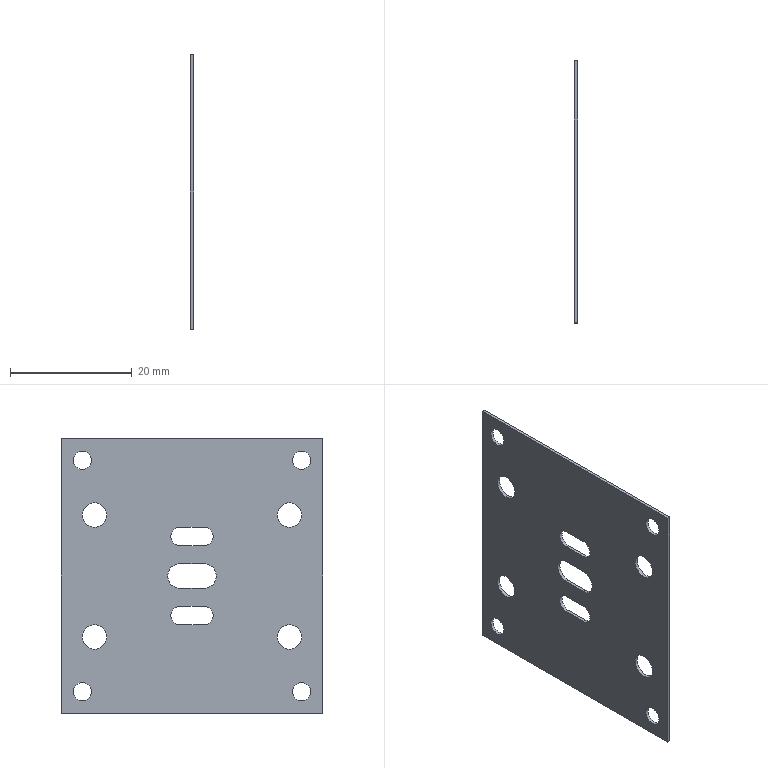Component | NX | 04__27 | 1 solid | 26 faces | volume 895 mm3 | cylinder 14 | plane 12 | commonest cylinder face diameters 3 x8 4 x6